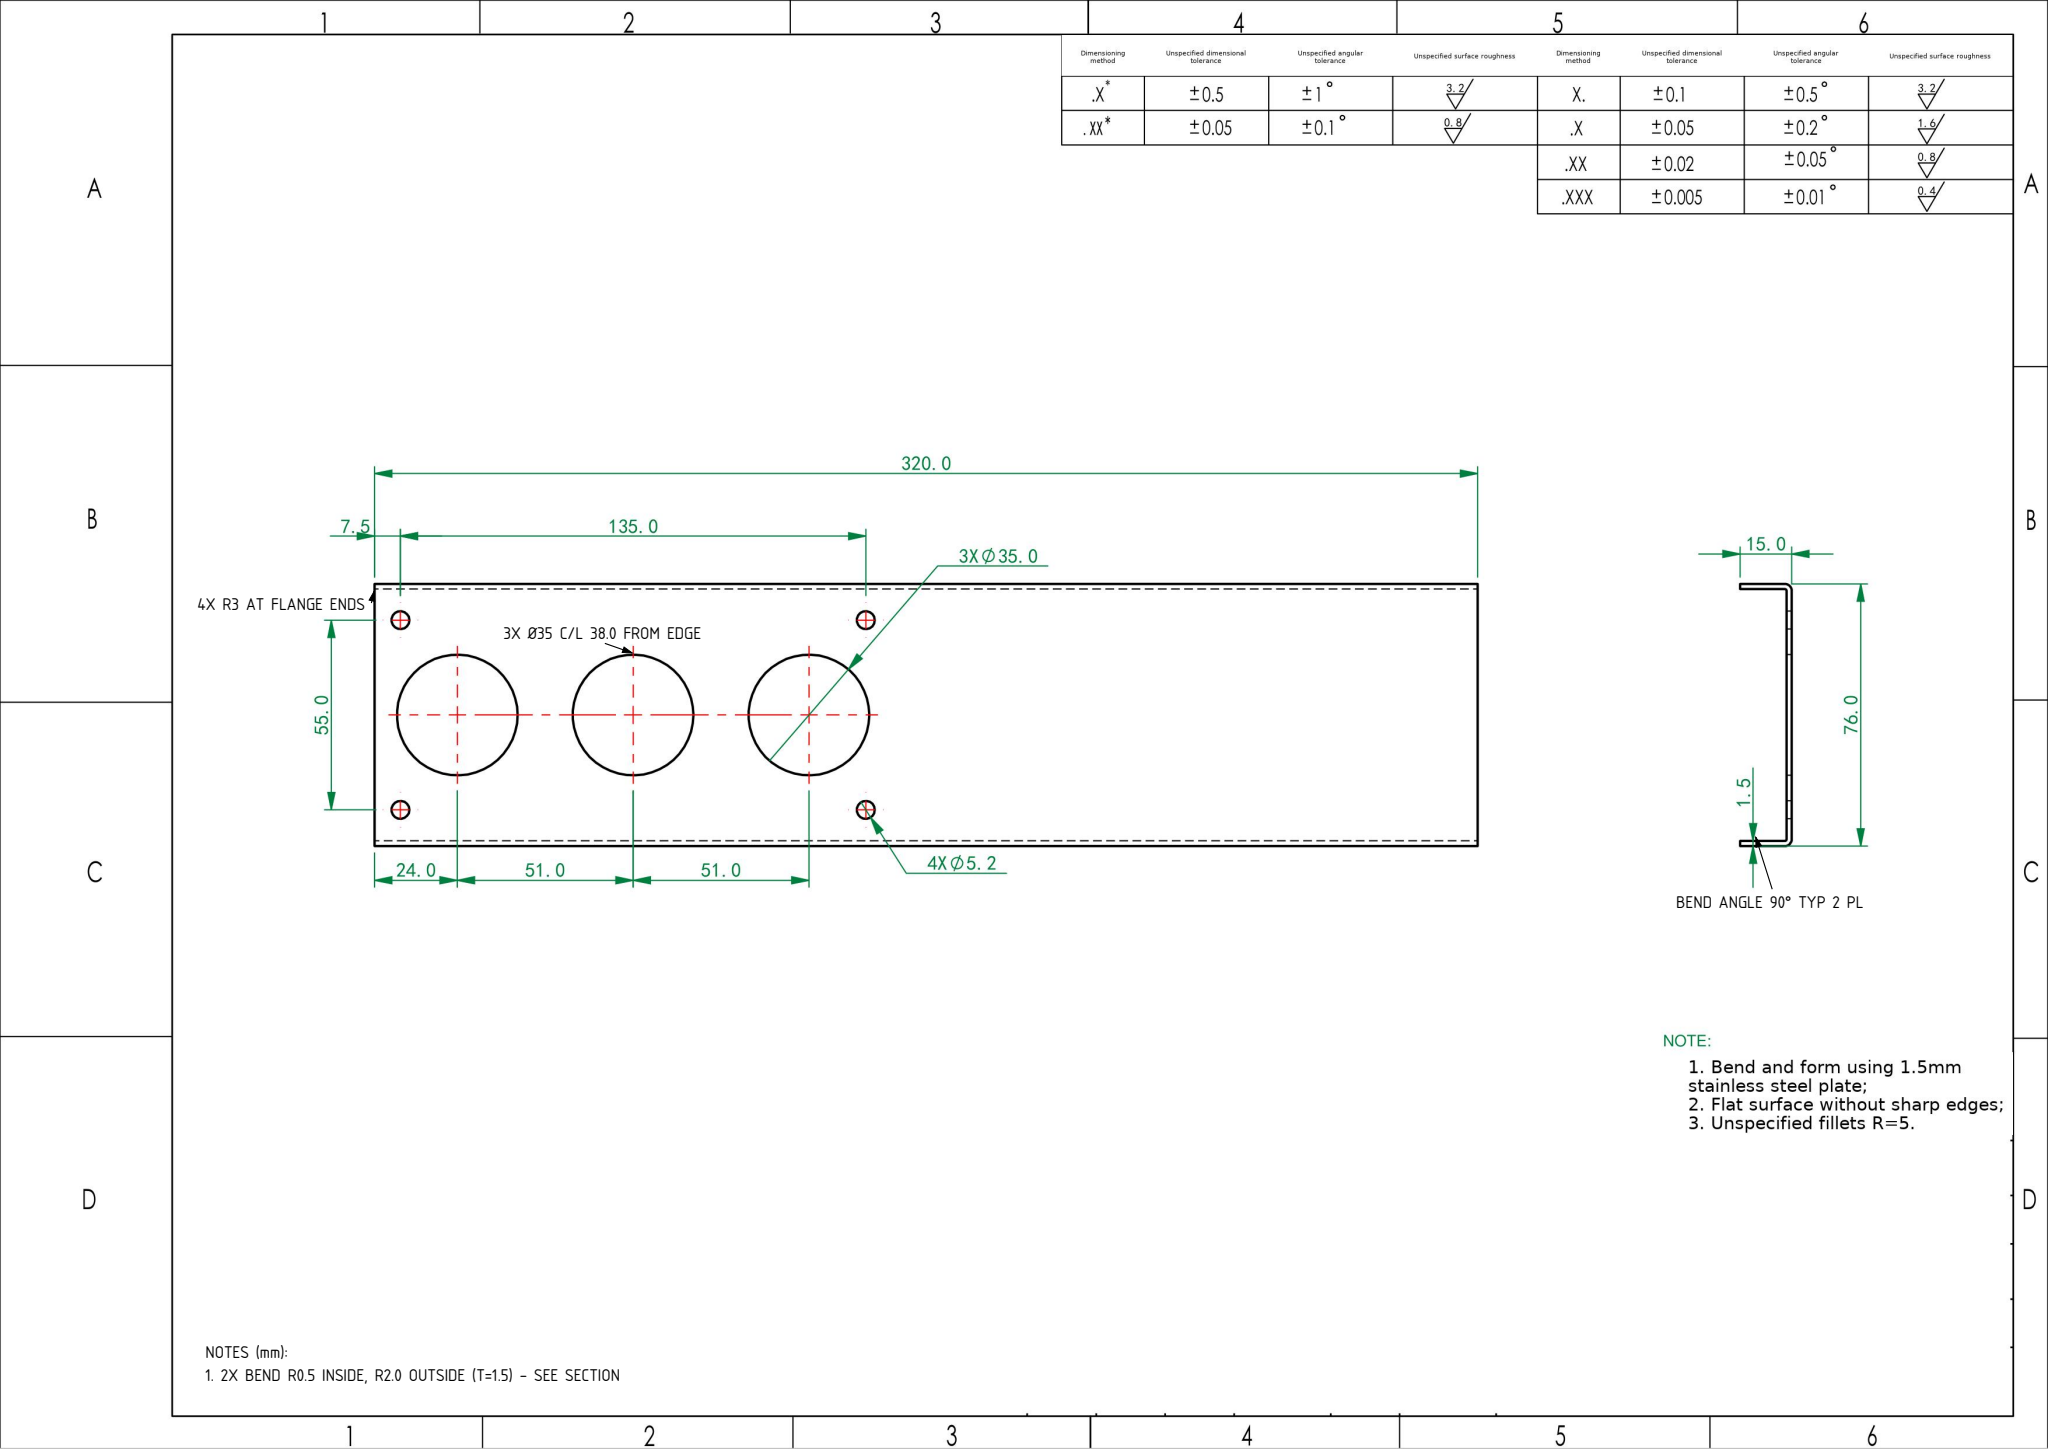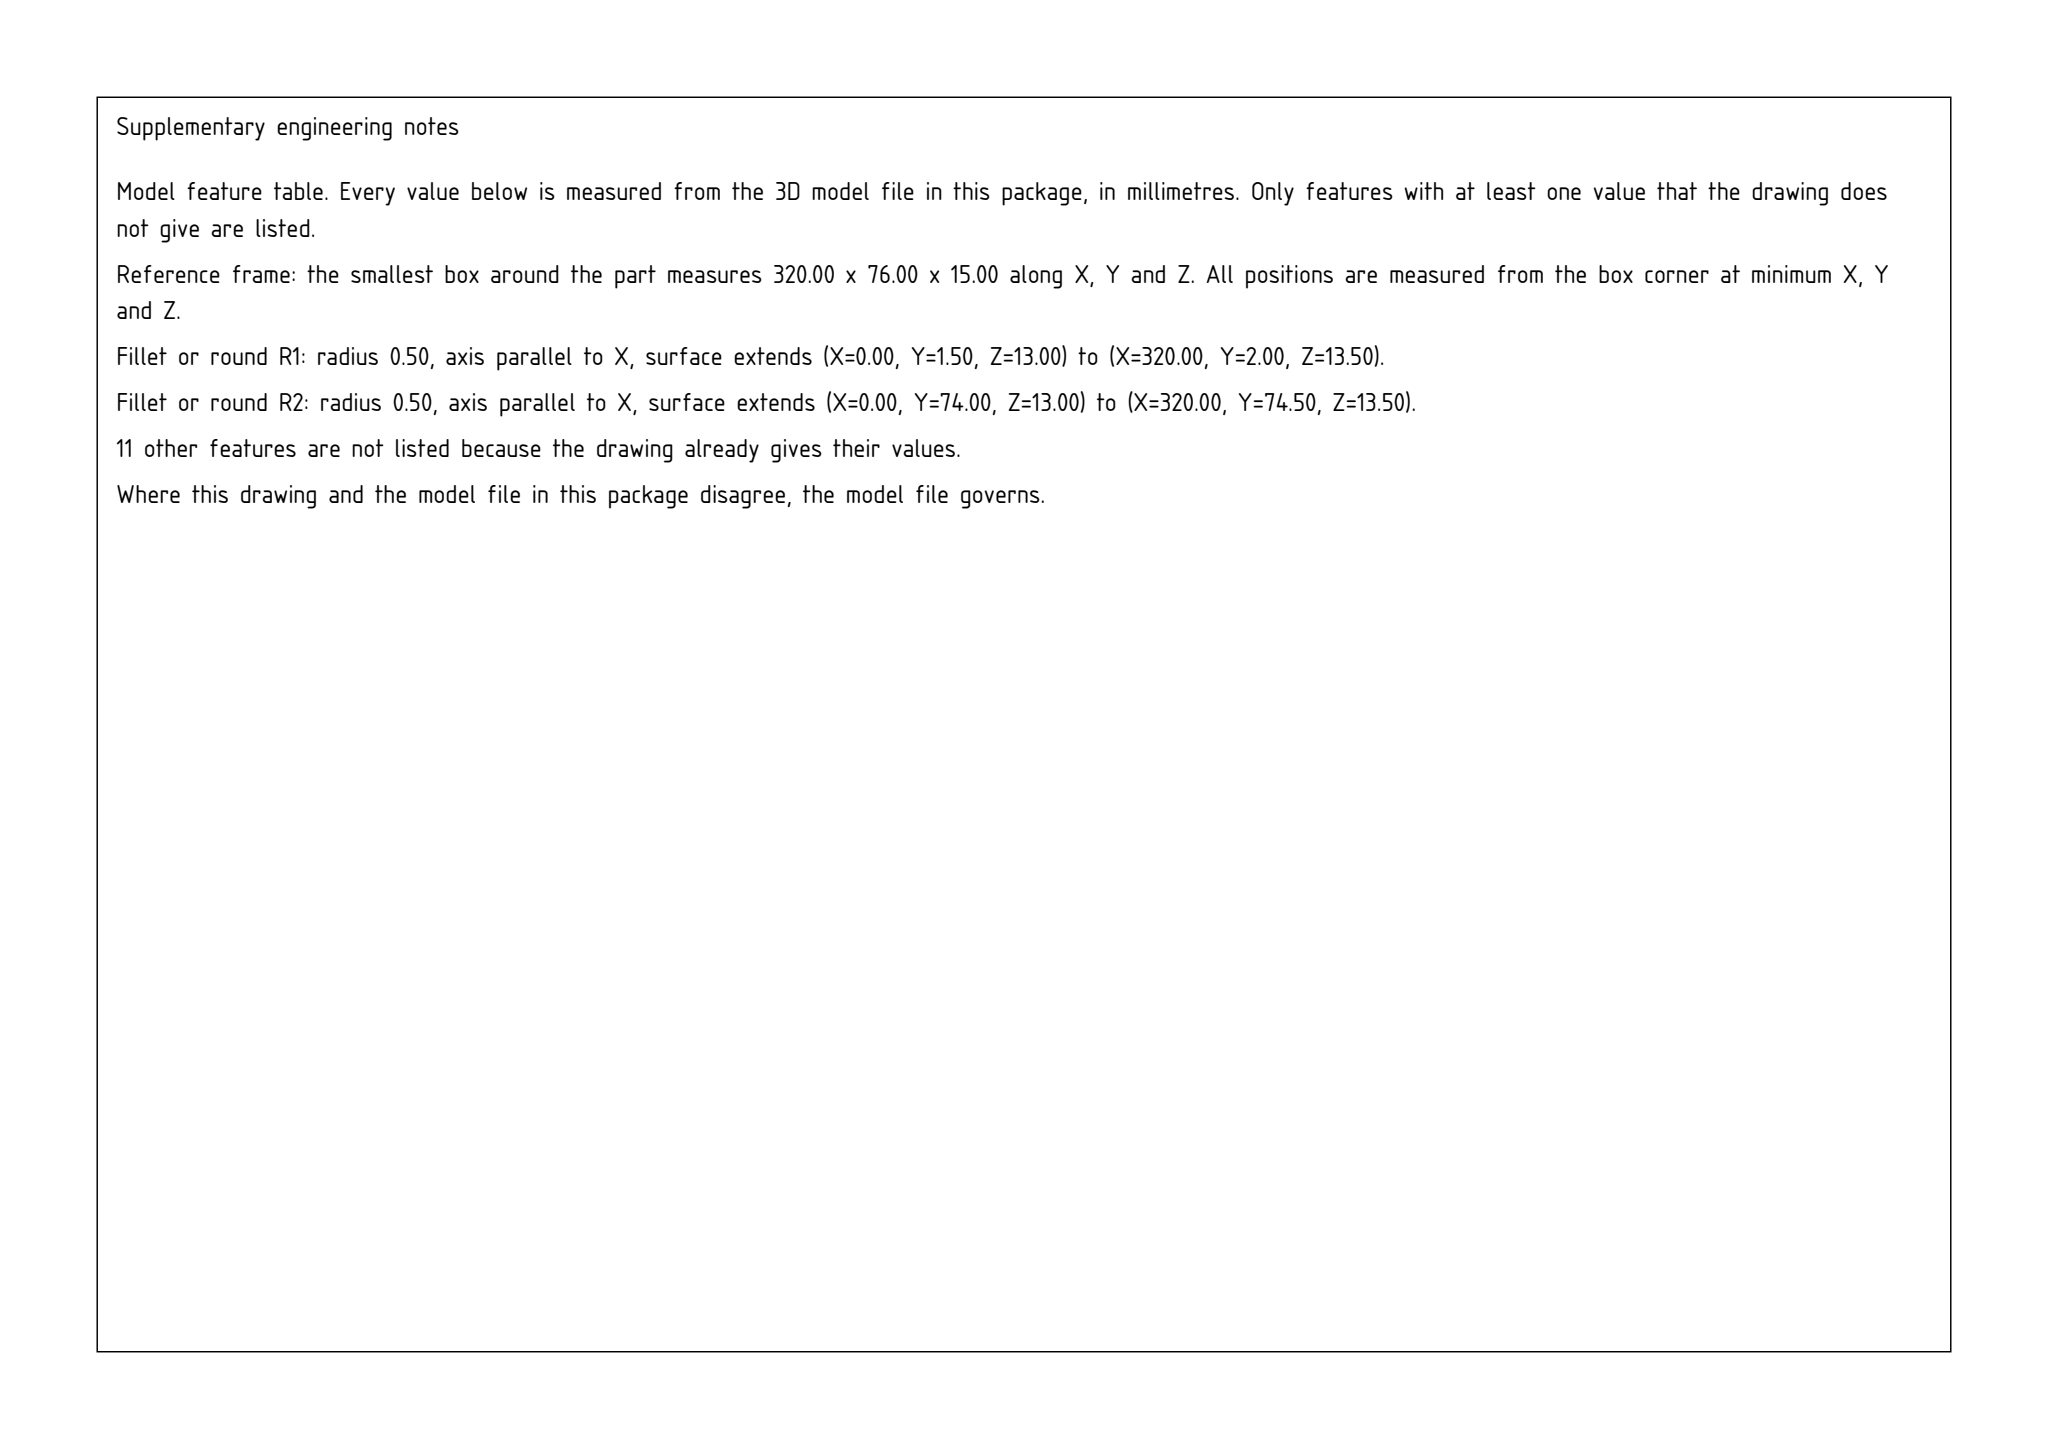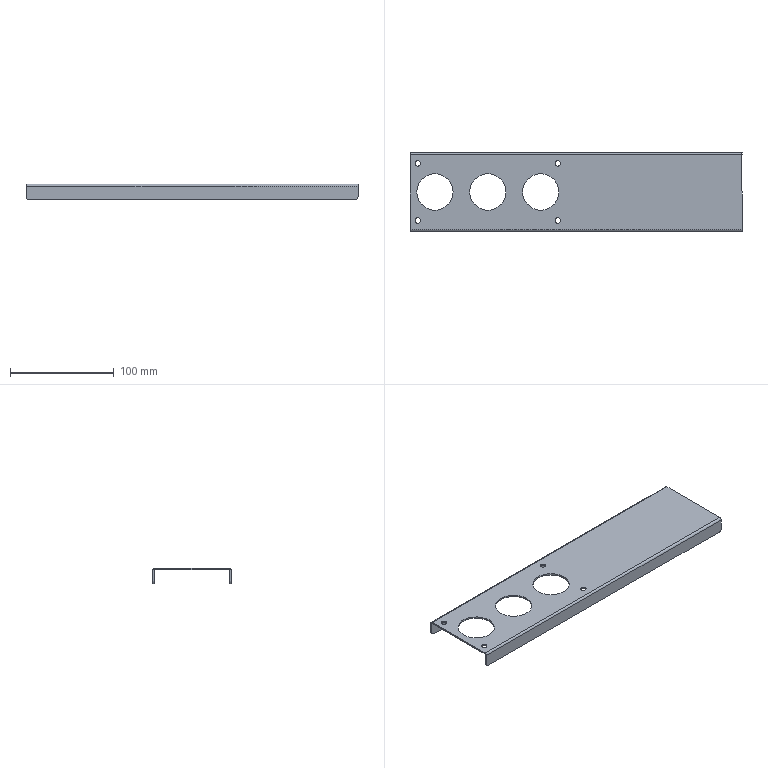Part | SolidWorks | mm | material 1.5mm stainless steel plate | 1 solid | 40 faces | box 320 x 76 x 15 mm | volume 44456 mm3 | cylinder 22 | plane 18 | commonest cylinder face diameters 5.2 x8 35 x6 6 x4 4 x2 1 x2
Drawing notes:
2X BEND R0.5 INSIDE, R2.0 OUTSIDE (T=1.5) - SEE SECTION | from the solid: cyl dia1.0 axis x @ y=2.0,z=13.0 & y=74.0,z=13.0 (inner R0.5); dia4.0 same axes (outer R2.0)
4X R3 AT FLANGE ENDS - OVERRIDES NOTE 3 | from the solid: cyl dia6.0 axis y @ x=3.0,z=3.0 and x=317.0,z=3.0, len 1.5
BEND ANGLE 90° TYP 2 PL | from the solid: planes z=0 (web) and z=13.5/15.0 flanges normal to y=0/76 walls; orthogonal faces x,y,z
3X Ø35 C/L 38.0 FROM EDGE; 4X Ø5.2 C/L 10.5 & 65.5 | from the solid: Ø35 holes at y=38.0; Ø5.2 holes at y=10.5 and y=65.5; part width 76.0